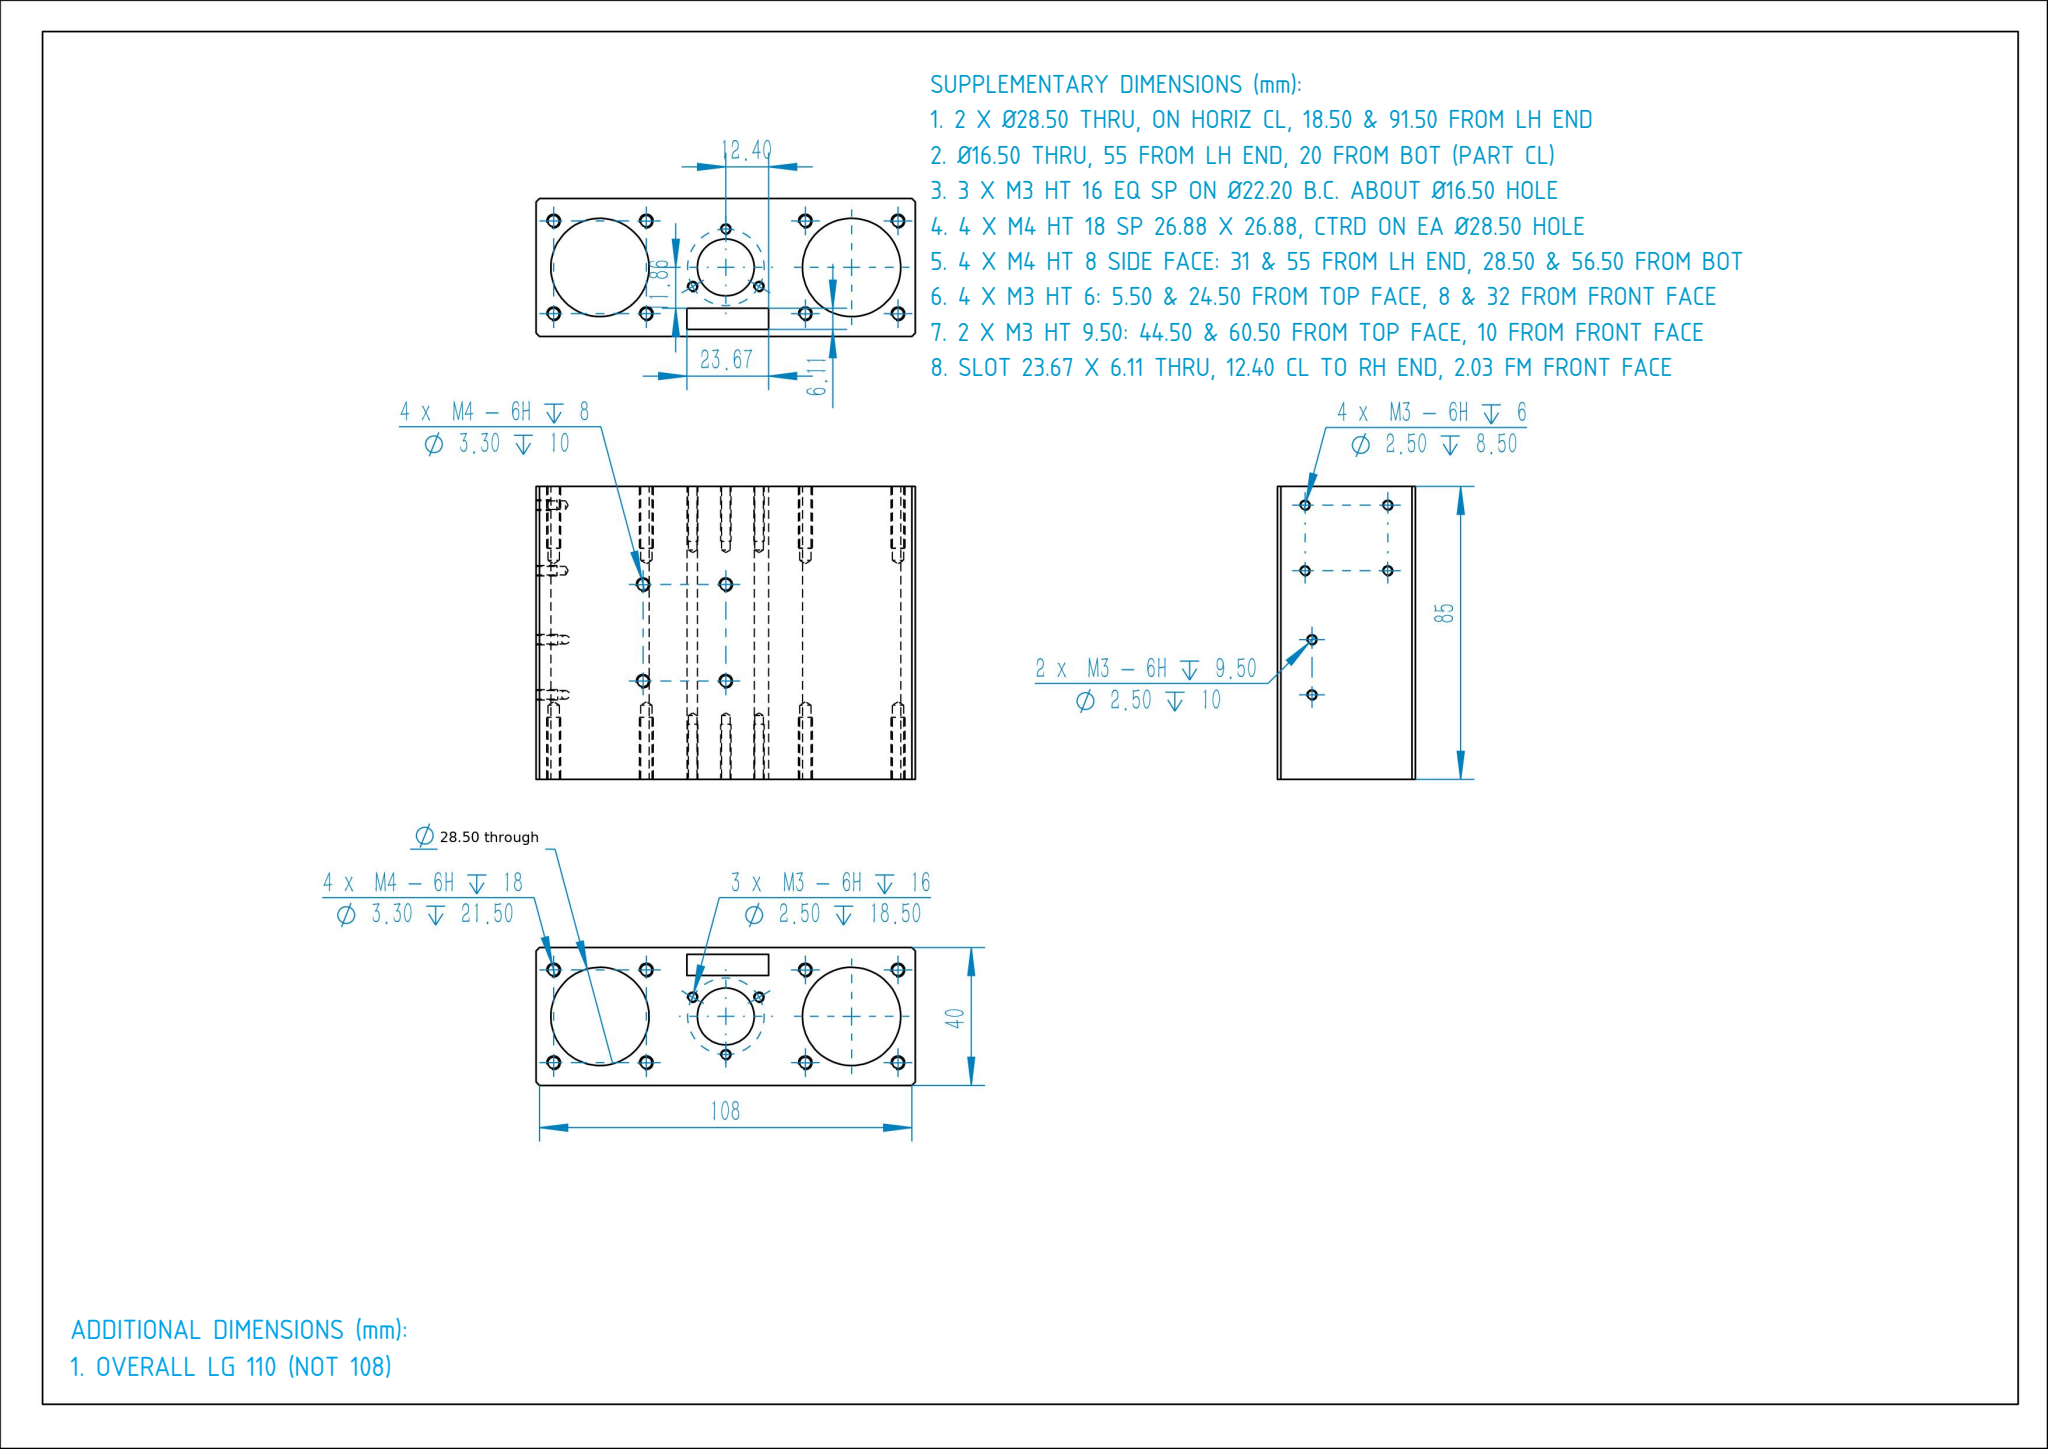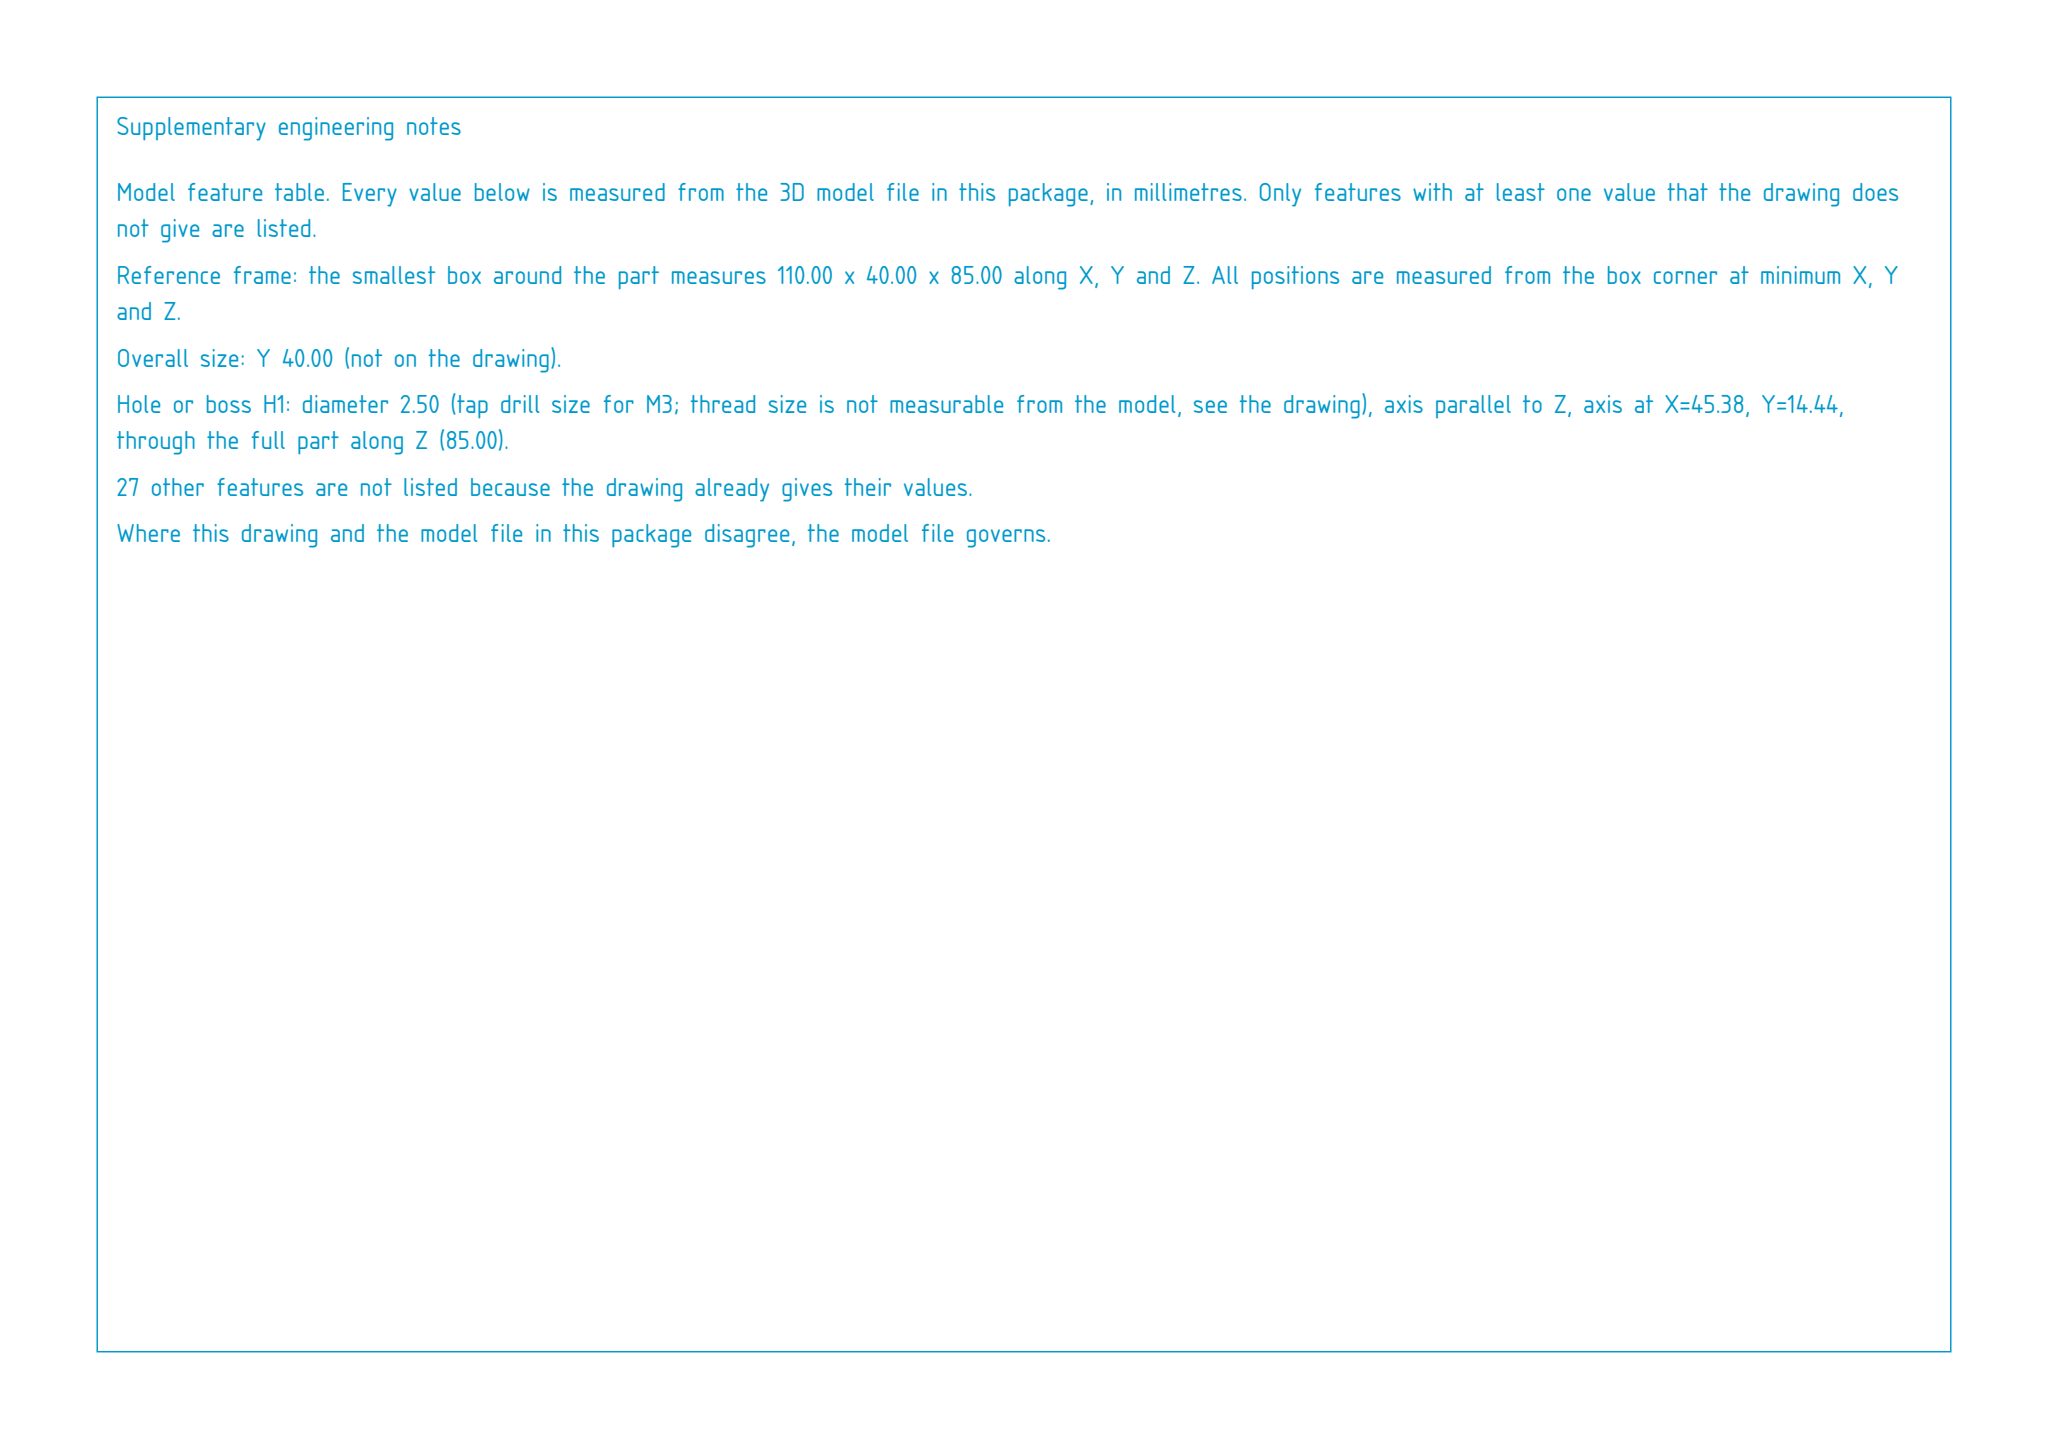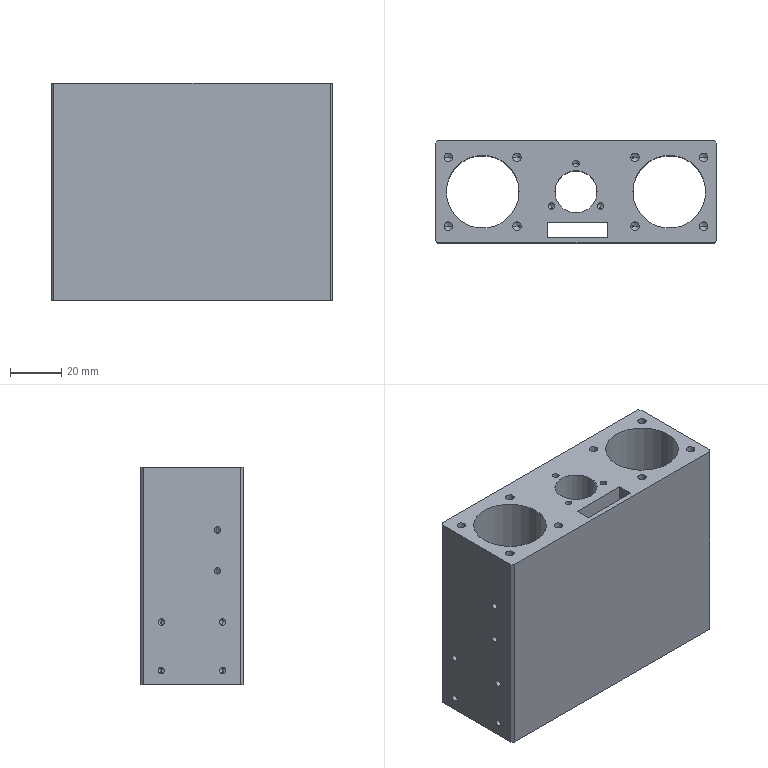Part | SolidWorks | mm | 1 solid | 146 faces | box 110 x 40 x 85 mm | volume 230772 mm3 | cylinder 72 | cone 60 | plane 14 | commonest cylinder face diameters 3.3 x40 2.5 x26 28.5 x4 16.5 x2
build123d program:
from build123d import *

# Parameters (mm, degrees)
SKETCH1_W            = 110
SKETCH1_H            = 85
BOSS_EXTRUDE1_DEPTH  = 20
SKETCH2_R            = 8.25
CUT_EXTRUDE1_DEPTH   = 104.199
CIRPATTERN2_COUNT    = 3
SKETCH8_R            = 14.25
CUT_EXTRUDE2_DEPTH   = 104.199
LPATTERN1_COUNT      = 2
LPATTERN1_PITCH      = 26.88
LPATTERN1_COUNT_DIR2 = 2
LPATTERN1_PITCH_DIR2 = 26.88
CHAMFER1_SIZE        = 1
CHAMFER2_SIZE        = 1
LPATTERN2_COUNT      = 2
LPATTERN2_PITCH      = 28
LPATTERN2_COUNT_DIR2 = 2
LPATTERN2_PITCH_DIR2 = 24
LPATTERN9_COUNT      = 2
LPATTERN9_PITCH      = 19
LPATTERN9_COUNT_DIR2 = 2
LPATTERN9_PITCH_DIR2 = 24
LPATTERN10_COUNT     = 2
LPATTERN10_PITCH     = 16
SKETCH19_W           = 23.669
SKETCH19_H           = 6.114
CUT_EXTRUDE3_DEPTH   = 170


with BuildPart() as part:
    # Sketch1 → Boss-Extrude1 (new, symmetric)
    with BuildSketch(Plane(origin=(0, 0, 0), x_dir=(1, 0, 0), z_dir=(0, 1, 0))):
        Rectangle(SKETCH1_W, SKETCH1_H)
    extrude(amount=BOSS_EXTRUDE1_DEPTH, both=True)

    # Sketch2 → Cut-Extrude1 (cut, through all)
    with BuildSketch(Plane.XY.offset(42.5)):
        Circle(SKETCH2_R)
    extrude(amount=-CUT_EXTRUDE1_DEPTH, mode=Mode.SUBTRACT)

    # Sketch6 → M3 Tapped Hole2 (revolve, cut)
    with BuildSketch(Plane(origin=(0, 11.11, -42.5), x_dir=(0, 1, 0), z_dir=(1, 0, 0))):
        Polygon((0, 0), (0, 19.251), (1.25, 18.5), (1.25, 0), align=None)
    m3_tapped_hole2 = revolve(axis=Axis((0, 11.11, -48.85), (0, 0, 1)), mode=Mode.SUBTRACT)

    # CirPattern2: M3 Tapped Hole2 ×3 about axis
    cirpattern2_axis = Axis((0, 0, 0), (0, 0, 1))
    for i in range(1, CIRPATTERN2_COUNT):
        add(m3_tapped_hole2.rotate(cirpattern2_axis, i * 360 / CIRPATTERN2_COUNT), mode=Mode.SUBTRACT)

    # Sketch8 → Cut-Extrude2 (cut, through all)
    with BuildSketch(Plane.XY.offset(42.5)):
        with Locations((-36.5, 0)):
            Circle(SKETCH8_R)
    cut_extrude2 = extrude(amount=-CUT_EXTRUDE2_DEPTH, mode=Mode.SUBTRACT)

    # Mirror1: Cut-Extrude2 across plane
    add(cut_extrude2.mirror(Plane(origin=(0, 0, 0), x_dir=(0, 0, 1), z_dir=(1, 0, 0))), mode=Mode.SUBTRACT)

    # Sketch9 → M4 Tapped Hole1 (revolve, cut)
    with BuildSketch(Plane(origin=(-49.94, 13.44, 42.5), x_dir=(0, -1, 0), z_dir=(1, 0, 0))):
        Polygon((0, 0), (0, 22.491), (1.65, 21.5), (1.65, 0), align=None)
    m4_tapped_hole1 = revolve(axis=Axis((-49.94, 13.44, 48.85), (0, 0, -1)), mode=Mode.SUBTRACT)

    # LPattern1: M4 Tapped Hole1 2 × 2
    with Locations(*[(i * LPATTERN1_PITCH, -j * LPATTERN1_PITCH_DIR2, 0) for i in range(LPATTERN1_COUNT) for j in range(LPATTERN1_COUNT_DIR2) if (i, j) != (0, 0)]):
        add(m4_tapped_hole1, mode=Mode.SUBTRACT)

    # Mirror2: M4 Tapped Hole1 across plane
    add(m4_tapped_hole1.mirror(Plane(origin=(0, 0, 0), x_dir=(0, 0, 1), z_dir=(1, 0, 0))), mode=Mode.SUBTRACT)

    # Mirror2 copy 1 sketch → Mirror2 copy 1 (revolve, cut)
    with BuildSketch(Plane(origin=(49.94, -13.44, 42.5), x_dir=(0, -1, 0), z_dir=(-1, 0, 0))):
        Polygon((0, 0), (0, -22.491), (1.65, -21.5), (1.65, 0), align=None)
    revolve(axis=Axis((49.94, -13.44, 48.85), (0, 0, 1)), mode=Mode.SUBTRACT)

    # Mirror2 copy 2 sketch → Mirror2 copy 2 (revolve, cut)
    with BuildSketch(Plane(origin=(23.06, 13.44, 42.5), x_dir=(0, -1, 0), z_dir=(-1, 0, 0))):
        Polygon((0, 0), (0, -22.491), (1.65, -21.5), (1.65, 0), align=None)
    revolve(axis=Axis((23.06, 13.44, 48.85), (0, 0, 1)), mode=Mode.SUBTRACT)

    # Mirror2 copy 3 sketch → Mirror2 copy 3 (revolve, cut)
    with BuildSketch(Plane(origin=(23.06, -13.44, 42.5), x_dir=(0, -1, 0), z_dir=(-1, 0, 0))):
        Polygon((0, 0), (0, -22.491), (1.65, -21.5), (1.65, 0), align=None)
    revolve(axis=Axis((23.06, -13.44, 48.85), (0, 0, 1)), mode=Mode.SUBTRACT)

    # Chamfer1
    chamfer1_edges = [part.edges().sort_by_distance(p)[0] for p in [
        (-55, 20, 0),
        (55, 20, 0),
    ]]
    chamfer(chamfer1_edges, length=CHAMFER1_SIZE)

    # Chamfer2
    chamfer2_edges = [part.edges().sort_by_distance(p)[0] for p in [
        (-55, -20, 0),
        (55, -20, 0),
    ]]
    chamfer(chamfer2_edges, length=CHAMFER2_SIZE)

    # Sketch11 → M4 Tapped Hole2 (revolve, cut)
    with BuildSketch(Plane(origin=(-24, 20, 14), x_dir=(0, 0, 1), z_dir=(1, 0, 0))):
        Polygon((0, 0), (0, 10.991), (1.65, 10), (1.65, 0), align=None)
    m4_tapped_hole2 = revolve(axis=Axis((-24, 26.35, 14), (0, -1, 0)), mode=Mode.SUBTRACT)

    # LPattern2: M4 Tapped Hole2 2 × 2
    with Locations(*[(j * LPATTERN2_PITCH_DIR2, 0, -i * LPATTERN2_PITCH) for i in range(LPATTERN2_COUNT) for j in range(LPATTERN2_COUNT_DIR2) if (i, j) != (0, 0)]):
        add(m4_tapped_hole2, mode=Mode.SUBTRACT)

    # Sketch15 → M3 Tapped Hole4 (revolve, cut)
    with BuildSketch(Plane(origin=(-55, 12, -37), x_dir=(0, 0, 1), z_dir=(0, 1, 0))):
        Polygon((0, 0), (0, 9.251), (1.25, 8.5), (1.25, 0), align=None)
    m3_tapped_hole4 = revolve(axis=Axis((-61.35, 12, -37), (1, 0, 0)), mode=Mode.SUBTRACT)

    # LPattern9: M3 Tapped Hole4 2 × 2
    with Locations(*[(0, -j * LPATTERN9_PITCH_DIR2, i * LPATTERN9_PITCH) for i in range(LPATTERN9_COUNT) for j in range(LPATTERN9_COUNT_DIR2) if (i, j) != (0, 0)]):
        add(m3_tapped_hole4, mode=Mode.SUBTRACT)

    # Sketch17 → M3 Tapped Hole5 (revolve, cut)
    with BuildSketch(Plane(origin=(-55, -10, 18), x_dir=(0, 0, 1), z_dir=(0, 1, 0))):
        Polygon((0, 0), (0, 10.751), (1.25, 10), (1.25, 0), align=None)
    m3_tapped_hole5 = revolve(axis=Axis((-61.35, -10, 18), (1, 0, 0)), mode=Mode.SUBTRACT)

    # LPattern10: M3 Tapped Hole5 ×2
    with Locations(*[(0, 0, -i * LPATTERN10_PITCH) for i in range(1, LPATTERN10_COUNT)]):
        add(m3_tapped_hole5, mode=Mode.SUBTRACT)

    # Mirror3: M4 Tapped Hole1 across plane
    add(m4_tapped_hole1.mirror(Plane.XY), mode=Mode.SUBTRACT)

    # Mirror3 copy 1 sketch → Mirror3 copy 1 (revolve, cut)
    with BuildSketch(Plane(origin=(-49.94, -13.44, -42.5), x_dir=(0, -1, 0), z_dir=(1, 0, 0))):
        Polygon((0, 0), (0, -22.491), (1.65, -21.5), (1.65, 0), align=None)
    revolve(axis=Axis((-49.94, -13.44, -48.85), (0, 0, -1)), mode=Mode.SUBTRACT)

    # Mirror3 copy 2 sketch → Mirror3 copy 2 (revolve, cut)
    with BuildSketch(Plane(origin=(-23.06, 13.44, -42.5), x_dir=(0, -1, 0), z_dir=(1, 0, 0))):
        Polygon((0, 0), (0, -22.491), (1.65, -21.5), (1.65, 0), align=None)
    revolve(axis=Axis((-23.06, 13.44, -48.85), (0, 0, -1)), mode=Mode.SUBTRACT)

    # Mirror3 copy 3 sketch → Mirror3 copy 3 (revolve, cut)
    with BuildSketch(Plane(origin=(-23.06, -13.44, -42.5), x_dir=(0, -1, 0), z_dir=(1, 0, 0))):
        Polygon((0, 0), (0, -22.491), (1.65, -21.5), (1.65, 0), align=None)
    revolve(axis=Axis((-23.06, -13.44, -48.85), (0, 0, -1)), mode=Mode.SUBTRACT)

    # Mirror3 copy 4 sketch → Mirror3 copy 4 (revolve, cut)
    with BuildSketch(Plane(origin=(49.94, 13.44, -42.5), x_dir=(0, -1, 0), z_dir=(-1, 0, 0))):
        Polygon((0, 0), (0, 22.491), (1.65, 21.5), (1.65, 0), align=None)
    revolve(axis=Axis((49.94, 13.44, -48.85), (0, 0, 1)), mode=Mode.SUBTRACT)

    # Mirror3 copy 5 sketch → Mirror3 copy 5 (revolve, cut)
    with BuildSketch(Plane(origin=(49.94, -13.44, -42.5), x_dir=(0, -1, 0), z_dir=(-1, 0, 0))):
        Polygon((0, 0), (0, 22.491), (1.65, 21.5), (1.65, 0), align=None)
    revolve(axis=Axis((49.94, -13.44, -48.85), (0, 0, 1)), mode=Mode.SUBTRACT)

    # Mirror3 copy 6 sketch → Mirror3 copy 6 (revolve, cut)
    with BuildSketch(Plane(origin=(23.06, 13.44, -42.5), x_dir=(0, -1, 0), z_dir=(-1, 0, 0))):
        Polygon((0, 0), (0, 22.491), (1.65, 21.5), (1.65, 0), align=None)
    revolve(axis=Axis((23.06, 13.44, -48.85), (0, 0, 1)), mode=Mode.SUBTRACT)

    # Mirror3 copy 7 sketch → Mirror3 copy 7 (revolve, cut)
    with BuildSketch(Plane(origin=(23.06, -13.44, -42.5), x_dir=(0, -1, 0), z_dir=(-1, 0, 0))):
        Polygon((0, 0), (0, 22.491), (1.65, 21.5), (1.65, 0), align=None)
    revolve(axis=Axis((23.06, -13.44, -48.85), (0, 0, 1)), mode=Mode.SUBTRACT)

    # Mirror4: M3 Tapped Hole2 across plane
    add(m3_tapped_hole2.mirror(Plane.XY), mode=Mode.SUBTRACT)

    # Mirror4 copy 1 sketch → Mirror4 copy 1 (revolve, cut)
    with BuildSketch(Plane(origin=(-9.622, -5.555, 42.5), x_dir=(-0.866, -0.5, 0), z_dir=(-0.5, 0.866, 0))):
        Polygon((0, 0), (0, -19.251), (1.25, -18.5), (1.25, 0), align=None)
    revolve(axis=Axis((-9.622, -5.555, 48.85), (0, 0, 1)), mode=Mode.SUBTRACT)

    # Mirror4 copy 2 sketch → Mirror4 copy 2 (revolve, cut)
    with BuildSketch(Plane(origin=(9.622, -5.555, 42.5), x_dir=(0.866, -0.5, 0), z_dir=(-0.5, -0.866, 0))):
        Polygon((0, 0), (0, -19.251), (1.25, -18.5), (1.25, 0), align=None)
    revolve(axis=Axis((9.622, -5.555, 48.85), (0, 0, 1)), mode=Mode.SUBTRACT)

    # Sketch19 → Cut-Extrude3 (cut)
    with BuildSketch(Plane.XY.offset(42.5)):
        with Locations((0.5675, -14.916)):
            Rectangle(SKETCH19_W, SKETCH19_H)
    extrude(amount=-CUT_EXTRUDE3_DEPTH, mode=Mode.SUBTRACT)


solid = part.part